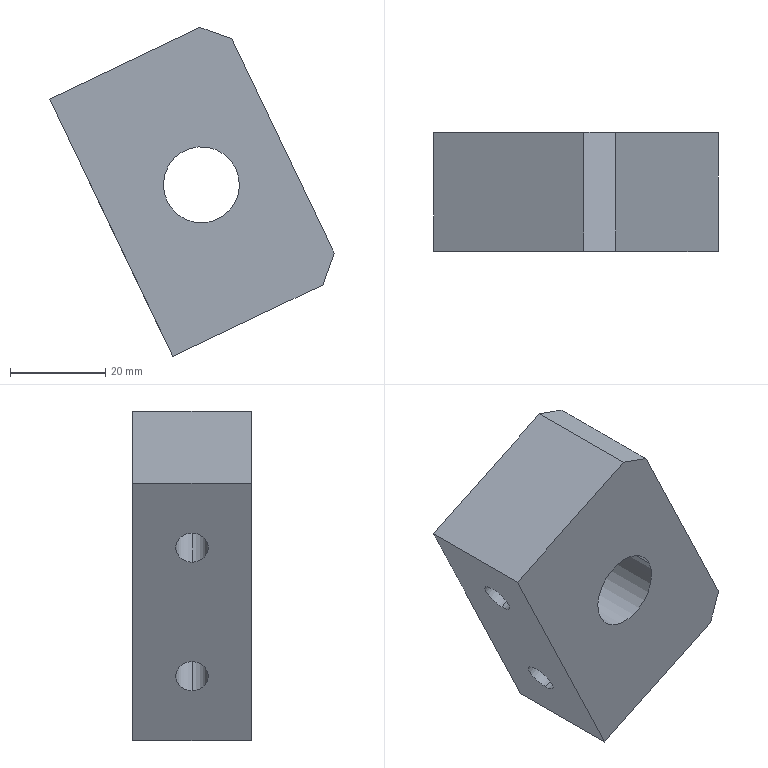Component | SolidWorks | FeedingPressingPlateAdjustmentBlock1-1-1 | 1 solid | 18 faces | box 59.83 x 25 x 69.23 mm | volume 52864 mm3 | plane 8 | cylinder 6 | cone 4 | commonest cylinder face diameters 6.8 x4 16 x2
build123d program:
from build123d import *

# Parameters (mm, degrees)
SKETCH1_W              = 60
SKETCH1_H              = 25
BOSS_EXTRUDE1_DEPTH    = 40
M8_TAPPED_HOLE1_D      = 6.8
M8_TAPPED_HOLE1_DEPTH  = 19.75
M8_TAPPED_HOLE1_TIP    = 2.043
M16_TAPPED_HOLE1_D     = 16
M16_TAPPED_HOLE1_DEPTH = 38
M16_TAPPED_HOLE1_TIP   = 4.807
CHAMFER1_SIZE          = 5


with BuildPart() as part:
    # Sketch1 → Boss-Extrude1 (new body)
    with BuildSketch(Plane.XY):
        with Locations((30, 12.5)):
            Rectangle(SKETCH1_W, SKETCH1_H)
    extrude(amount=BOSS_EXTRUDE1_DEPTH)

    # M8 Tapped Hole1
    with Locations(Plane(origin=(45, 12.5, 0), x_dir=(-1, 0, 0), z_dir=(0, 0, -1))):
        with Locations((0, 0), (30, 0)):
            Hole(M8_TAPPED_HOLE1_D / 2, depth=M8_TAPPED_HOLE1_DEPTH)
            with Locations((0, 0, -(M8_TAPPED_HOLE1_DEPTH + M8_TAPPED_HOLE1_TIP / 2))):  # 118° drill point
                Cone(0, M8_TAPPED_HOLE1_D / 2, M8_TAPPED_HOLE1_TIP, mode=Mode.SUBTRACT)

    # M16 Tapped Hole1
    with Locations(Plane(origin=(30, 25, 21), x_dir=(0, 0, 1), z_dir=(0, 1, 0))):
        with Locations((0, 0)):
            Hole(M16_TAPPED_HOLE1_D / 2, depth=M16_TAPPED_HOLE1_DEPTH)
            with Locations((0, 0, -(M16_TAPPED_HOLE1_DEPTH + M16_TAPPED_HOLE1_TIP / 2))):  # 118° drill point
                Cone(0, M16_TAPPED_HOLE1_D / 2, M16_TAPPED_HOLE1_TIP, mode=Mode.SUBTRACT)

    # Chamfer1
    chamfer1_edges = [part.edges().sort_by_distance(p)[0] for p in [
        (60, 12.5, 40),
        (0, 12.5, 40),
    ]]
    chamfer(chamfer1_edges, length=CHAMFER1_SIZE)


solid = part.part

# Placed as in the assembly
solid = solid.moved(Location((-27.022, 360, 606.201), (0, 64.419, 0)))
STEP:
#1=COLOUR_RGB('',0.7922,0.8196,0.9333);
#2=FILL_AREA_STYLE_COLOUR('',#1);
#3=FILL_AREA_STYLE('',(#2));
#4=SURFACE_STYLE_FILL_AREA(#3);
#5=SURFACE_SIDE_STYLE('',(#4));
#6=SURFACE_STYLE_USAGE(.BOTH.,#5);
#7=PRESENTATION_STYLE_ASSIGNMENT((#6));
#8=CARTESIAN_POINT('',(-0.09223,14.173,23.022));
#9=VERTEX_POINT('',#8);
#10=CARTESIAN_POINT('',(0.4759,14.173,23.294));
#11=VERTEX_POINT('',#10);
#12=CARTESIAN_POINT('',(0.1919,14.173,23.158));
#13=DIRECTION('',(0.,1.,-0.));
#14=DIRECTION('',(0.902,0.,0.4318));
#15=AXIS2_PLACEMENT_3D('',#12,#13,#14);
#16=CIRCLE('',#15,0.315);
#17=EDGE_CURVE('',#9,#11,#16,.T.);
#18=ORIENTED_EDGE('',*,*,#17,.F.);
#19=CARTESIAN_POINT('',(-0.09223,15.157,23.022));
#20=VERTEX_POINT('',#19);
#21=CARTESIAN_POINT('',(-0.09223,15.157,23.022));
#22=DIRECTION('',(0.,1.,-0.));
#23=VECTOR('',#22,39.37);
#24=LINE('',#21,#23);
#25=EDGE_CURVE('',#9,#20,#24,.T.);
#26=ORIENTED_EDGE('',*,*,#25,.T.);
#27=CARTESIAN_POINT('',(0.4759,15.157,23.294));
#28=VERTEX_POINT('',#27);
#29=CARTESIAN_POINT('',(0.1919,15.157,23.158));
#30=DIRECTION('',(0.,1.,-0.));
#31=DIRECTION('',(0.902,0.,0.4318));
#32=AXIS2_PLACEMENT_3D('',#29,#30,#31);
#33=CIRCLE('',#32,0.315);
#34=EDGE_CURVE('',#20,#28,#33,.T.);
#35=ORIENTED_EDGE('',*,*,#34,.T.);
#36=CARTESIAN_POINT('',(0.4759,15.157,23.294));
#37=DIRECTION('',(0.,1.,-0.));
#38=VECTOR('',#37,39.37);
#39=LINE('',#36,#38);
#40=EDGE_CURVE('',#11,#28,#39,.T.);
#41=ORIENTED_EDGE('',*,*,#40,.F.);
#42=EDGE_LOOP('',(#18,#26,#35,#41));
#43=FACE_OUTER_BOUND('',#42,.T.);
#44=CARTESIAN_POINT('',(0.1919,15.157,23.158));
#45=DIRECTION('',(0.,1.,-0.));
#46=DIRECTION('',(0.902,0.,0.4318));
#47=AXIS2_PLACEMENT_3D('',#44,#45,#46);
#48=CYLINDRICAL_SURFACE('',#47,0.315);
#49=ADVANCED_FACE('',(#43),#48,.F.);
#50=CARTESIAN_POINT('',(0.4603,14.665,22.483));
#51=VERTEX_POINT('',#50);
#52=CARTESIAN_POINT('',(0.3447,14.665,22.725));
#53=VERTEX_POINT('',#52);
#54=CARTESIAN_POINT('',(0.4025,14.665,22.604));
#55=DIRECTION('',(-0.902,0.,-0.4318));
#56=DIRECTION('',(-0.4318,0.,0.902));
#57=AXIS2_PLACEMENT_3D('',#54,#55,#56);
#58=CIRCLE('',#57,0.1339);
#59=EDGE_CURVE('',#51,#53,#58,.T.);
#60=ORIENTED_EDGE('',*,*,#59,.F.);
#61=CARTESIAN_POINT('',(-0.2411,14.665,22.147));
#62=VERTEX_POINT('',#61);
#63=CARTESIAN_POINT('',(-0.2411,14.665,22.147));
#64=DIRECTION('',(-0.902,0.,-0.4318));
#65=VECTOR('',#64,39.37);
#66=LINE('',#63,#65);
#67=EDGE_CURVE('',#51,#62,#66,.T.);
#68=ORIENTED_EDGE('',*,*,#67,.T.);
#69=CARTESIAN_POINT('',(-0.3567,14.665,22.389));
#70=VERTEX_POINT('',#69);
#71=CARTESIAN_POINT('',(-0.2989,14.665,22.268));
#72=DIRECTION('',(-0.902,0.,-0.4318));
#73=DIRECTION('',(-0.4318,0.,0.902));
#74=AXIS2_PLACEMENT_3D('',#71,#72,#73);
#75=CIRCLE('',#74,0.1339);
#76=EDGE_CURVE('',#62,#70,#75,.T.);
#77=ORIENTED_EDGE('',*,*,#76,.T.);
#78=CARTESIAN_POINT('',(-0.3567,14.665,22.389));
#79=DIRECTION('',(-0.902,0.,-0.4318));
#80=VECTOR('',#79,39.37);
#81=LINE('',#78,#80);
#82=EDGE_CURVE('',#53,#70,#81,.T.);
#83=ORIENTED_EDGE('',*,*,#82,.F.);
#84=EDGE_LOOP('',(#60,#68,#77,#83));
#85=FACE_OUTER_BOUND('',#84,.T.);
#86=CARTESIAN_POINT('',(-0.2989,14.665,22.268));
#87=DIRECTION('',(-0.902,0.,-0.4318));
#88=DIRECTION('',(-0.4318,0.,0.902));
#89=AXIS2_PLACEMENT_3D('',#86,#87,#88);
#90=CYLINDRICAL_SURFACE('',#89,0.1339);
#91=ADVANCED_FACE('',(#85),#90,.F.);
#92=CARTESIAN_POINT('',(0.475,14.665,22.639));
#93=VERTEX_POINT('',#92);
#94=CARTESIAN_POINT('',(0.3447,14.665,22.725));
#95=DIRECTION('',(-0.8347,0.,0.5508));
#96=VECTOR('',#95,39.37);
#97=LINE('',#94,#96);
#98=EDGE_CURVE('',#93,#53,#97,.T.);
#99=ORIENTED_EDGE('',*,*,#98,.F.);
#100=CARTESIAN_POINT('',(0.4603,14.665,22.483));
#101=DIRECTION('',(-0.09444,-0.,-0.9955));
#102=VECTOR('',#101,39.37);
#103=LINE('',#100,#102);
#104=EDGE_CURVE('',#93,#51,#103,.T.);
#105=ORIENTED_EDGE('',*,*,#104,.T.);
#106=ORIENTED_EDGE('',*,*,#59,.T.);
#107=EDGE_LOOP('',(#99,#105,#106));
#108=FACE_OUTER_BOUND('',#107,.T.);
#109=CARTESIAN_POINT('',(0.4025,14.665,22.604));
#110=DIRECTION('',(-0.902,0.,-0.4318));
#111=DIRECTION('',(-0.4318,0.,0.902));
#112=AXIS2_PLACEMENT_3D('',#109,#110,#111);
#113=CONICAL_SURFACE('',#112,0.1339,1.03);
#114=ADVANCED_FACE('',(#108),#113,.F.);
#115=CARTESIAN_POINT('',(-0.04972,14.665,23.549));
#116=VERTEX_POINT('',#115);
#117=CARTESIAN_POINT('',(-0.1653,14.665,23.79));
#118=VERTEX_POINT('',#117);
#119=CARTESIAN_POINT('',(-0.1075,14.665,23.669));
#120=DIRECTION('',(-0.902,0.,-0.4318));
#121=DIRECTION('',(-0.4318,0.,0.902));
#122=AXIS2_PLACEMENT_3D('',#119,#120,#121);
#123=CIRCLE('',#122,0.1339);
#124=EDGE_CURVE('',#116,#118,#123,.T.);
#125=ORIENTED_EDGE('',*,*,#124,.F.);
#126=CARTESIAN_POINT('',(-0.7511,14.665,23.213));
#127=VERTEX_POINT('',#126);
#128=CARTESIAN_POINT('',(-0.7511,14.665,23.213));
#129=DIRECTION('',(-0.902,0.,-0.4318));
#130=VECTOR('',#129,39.37);
#131=LINE('',#128,#130);
#132=EDGE_CURVE('',#116,#127,#131,.T.);
#133=ORIENTED_EDGE('',*,*,#132,.T.);
#134=CARTESIAN_POINT('',(-0.8667,14.665,23.454));
#135=VERTEX_POINT('',#134);
#136=CARTESIAN_POINT('',(-0.8089,14.665,23.334));
#137=DIRECTION('',(-0.902,0.,-0.4318));
#138=DIRECTION('',(-0.4318,0.,0.902));
#139=AXIS2_PLACEMENT_3D('',#136,#137,#138);
#140=CIRCLE('',#139,0.1339);
#141=EDGE_CURVE('',#127,#135,#140,.T.);
#142=ORIENTED_EDGE('',*,*,#141,.T.);
#143=CARTESIAN_POINT('',(-0.8667,14.665,23.454));
#144=DIRECTION('',(-0.902,0.,-0.4318));
#145=VECTOR('',#144,39.37);
#146=LINE('',#143,#145);
#147=EDGE_CURVE('',#118,#135,#146,.T.);
#148=ORIENTED_EDGE('',*,*,#147,.F.);
#149=EDGE_LOOP('',(#125,#133,#142,#148));
#150=FACE_OUTER_BOUND('',#149,.T.);
#151=CARTESIAN_POINT('',(-0.8089,14.665,23.334));
#152=DIRECTION('',(-0.902,0.,-0.4318));
#153=DIRECTION('',(-0.4318,0.,0.902));
#154=AXIS2_PLACEMENT_3D('',#151,#152,#153);
#155=CYLINDRICAL_SURFACE('',#154,0.1339);
#156=ADVANCED_FACE('',(#150),#155,.F.);
#157=CARTESIAN_POINT('',(-0.03498,14.665,23.704));
#158=VERTEX_POINT('',#157);
#159=CARTESIAN_POINT('',(-0.1653,14.665,23.79));
#160=DIRECTION('',(-0.8347,0.,0.5508));
#161=VECTOR('',#160,39.37);
#162=LINE('',#159,#161);
#163=EDGE_CURVE('',#158,#118,#162,.T.);
#164=ORIENTED_EDGE('',*,*,#163,.F.);
#165=CARTESIAN_POINT('',(-0.04972,14.665,23.549));
#166=DIRECTION('',(-0.09444,-0.,-0.9955));
#167=VECTOR('',#166,39.37);
#168=LINE('',#165,#167);
#169=EDGE_CURVE('',#158,#116,#168,.T.);
#170=ORIENTED_EDGE('',*,*,#169,.T.);
#171=ORIENTED_EDGE('',*,*,#124,.T.);
#172=EDGE_LOOP('',(#164,#170,#171));
#173=FACE_OUTER_BOUND('',#172,.T.);
#174=CARTESIAN_POINT('',(-0.1075,14.665,23.669));
#175=DIRECTION('',(-0.902,0.,-0.4318));
#176=DIRECTION('',(-0.4318,0.,0.902));
#177=AXIS2_PLACEMENT_3D('',#174,#175,#176);
#178=CONICAL_SURFACE('',#177,0.1339,1.03);
#179=ADVANCED_FACE('',(#173),#178,.F.);
#180=CARTESIAN_POINT('',(0.179,14.173,24.461));
#181=VERTEX_POINT('',#180);
#182=CARTESIAN_POINT('',(-1.064,14.173,23.866));
#183=VERTEX_POINT('',#182);
#184=CARTESIAN_POINT('',(0.3566,14.173,24.546));
#185=DIRECTION('',(-0.902,0.,-0.4318));
#186=VECTOR('',#185,39.37);
#187=LINE('',#184,#186);
#188=EDGE_CURVE('',#181,#183,#187,.T.);
#189=ORIENTED_EDGE('',*,*,#188,.F.);
#190=CARTESIAN_POINT('',(0.179,15.157,24.461));
#191=VERTEX_POINT('',#190);
#192=CARTESIAN_POINT('',(0.179,14.173,24.461));
#193=DIRECTION('',(0.,1.,-0.));
#194=VECTOR('',#193,39.37);
#195=LINE('',#192,#194);
#196=EDGE_CURVE('',#181,#191,#195,.T.);
#197=ORIENTED_EDGE('',*,*,#196,.T.);
#198=CARTESIAN_POINT('',(-1.064,15.157,23.866));
#199=VERTEX_POINT('',#198);
#200=CARTESIAN_POINT('',(0.3566,15.157,24.546));
#201=DIRECTION('',(-0.902,0.,-0.4318));
#202=VECTOR('',#201,39.37);
#203=LINE('',#200,#202);
#204=EDGE_CURVE('',#191,#199,#203,.T.);
#205=ORIENTED_EDGE('',*,*,#204,.T.);
#206=CARTESIAN_POINT('',(-1.064,14.173,23.866));
#207=DIRECTION('',(-0.,-1.,0.));
#208=VECTOR('',#207,39.37);
#209=LINE('',#206,#208);
#210=EDGE_CURVE('',#199,#183,#209,.T.);
#211=ORIENTED_EDGE('',*,*,#210,.T.);
#212=EDGE_LOOP('',(#189,#197,#205,#211));
#213=FACE_OUTER_BOUND('',#212,.T.);
#214=CARTESIAN_POINT('',(0.3566,14.173,24.546));
#215=DIRECTION('',(0.4318,-0.,-0.902));
#216=DIRECTION('',(-0.902,0.,-0.4318));
#217=AXIS2_PLACEMENT_3D('',#214,#215,#216);
#218=PLANE('',#217);
#219=ADVANCED_FACE('',(#213),#218,.F.);
#220=CARTESIAN_POINT('',(0.1919,14.173,23.158));
#221=DIRECTION('',(0.,1.,-0.));
#222=DIRECTION('',(0.902,0.,0.4318));
#223=AXIS2_PLACEMENT_3D('',#220,#221,#222);
#224=CIRCLE('',#223,0.315);
#225=EDGE_CURVE('',#11,#9,#224,.T.);
#226=ORIENTED_EDGE('',*,*,#225,.T.);
#227=ORIENTED_EDGE('',*,*,#17,.T.);
#228=EDGE_LOOP('',(#226,#227));
#229=FACE_BOUND('',#228,.T.);
#230=CARTESIAN_POINT('',(1.199,14.173,22.33));
#231=VERTEX_POINT('',#230);
#232=CARTESIAN_POINT('',(-0.04389,14.173,21.736));
#233=VERTEX_POINT('',#232);
#234=CARTESIAN_POINT('',(1.377,14.173,22.415));
#235=DIRECTION('',(-0.902,0.,-0.4318));
#236=VECTOR('',#235,39.37);
#237=LINE('',#234,#236);
#238=EDGE_CURVE('',#231,#233,#237,.T.);
#239=ORIENTED_EDGE('',*,*,#238,.F.);
#240=CARTESIAN_POINT('',(1.292,14.173,22.593));
#241=VERTEX_POINT('',#240);
#242=CARTESIAN_POINT('',(1.292,14.173,22.593));
#243=DIRECTION('',(0.3325,0.,0.9431));
#244=VECTOR('',#243,39.37);
#245=LINE('',#242,#244);
#246=EDGE_CURVE('',#231,#241,#245,.T.);
#247=ORIENTED_EDGE('',*,*,#246,.T.);
#248=CARTESIAN_POINT('',(0.4416,14.173,24.369));
#249=VERTEX_POINT('',#248);
#250=CARTESIAN_POINT('',(0.3566,14.173,24.546));
#251=DIRECTION('',(0.4318,-0.,-0.902));
#252=VECTOR('',#251,39.37);
#253=LINE('',#250,#252);
#254=EDGE_CURVE('',#249,#241,#253,.T.);
#255=ORIENTED_EDGE('',*,*,#254,.F.);
#256=CARTESIAN_POINT('',(0.4416,14.173,24.369));
#257=DIRECTION('',(-0.9431,0.,0.3325));
#258=VECTOR('',#257,39.37);
#259=LINE('',#256,#258);
#260=EDGE_CURVE('',#249,#181,#259,.T.);
#261=ORIENTED_EDGE('',*,*,#260,.T.);
#262=ORIENTED_EDGE('',*,*,#188,.T.);
#263=CARTESIAN_POINT('',(-1.064,14.173,23.866));
#264=DIRECTION('',(0.4318,-0.,-0.902));
#265=VECTOR('',#264,39.37);
#266=LINE('',#263,#265);
#267=EDGE_CURVE('',#183,#233,#266,.T.);
#268=ORIENTED_EDGE('',*,*,#267,.T.);
#269=EDGE_LOOP('',(#239,#247,#255,#261,#262,#268));
#270=FACE_OUTER_BOUND('',#269,.T.);
#271=CARTESIAN_POINT('',(0.3566,14.173,24.546));
#272=DIRECTION('',(0.,1.,-0.));
#273=DIRECTION('',(0.902,-0.,0.4318));
#274=AXIS2_PLACEMENT_3D('',#271,#272,#273);
#275=PLANE('',#274);
#276=ADVANCED_FACE('',(#229,#270),#275,.F.);
#277=CARTESIAN_POINT('',(1.199,15.157,22.33));
#278=VERTEX_POINT('',#277);
#279=CARTESIAN_POINT('',(-0.04389,15.157,21.736));
#280=VERTEX_POINT('',#279);
#281=CARTESIAN_POINT('',(1.377,15.157,22.415));
#282=DIRECTION('',(-0.902,0.,-0.4318));
#283=VECTOR('',#282,39.37);
#284=LINE('',#281,#283);
#285=EDGE_CURVE('',#278,#280,#284,.T.);
#286=ORIENTED_EDGE('',*,*,#285,.F.);
#287=CARTESIAN_POINT('',(1.199,14.173,22.33));
#288=DIRECTION('',(-0.,-1.,0.));
#289=VECTOR('',#288,39.37);
#290=LINE('',#287,#289);
#291=EDGE_CURVE('',#278,#231,#290,.T.);
#292=ORIENTED_EDGE('',*,*,#291,.T.);
#293=ORIENTED_EDGE('',*,*,#238,.T.);
#294=CARTESIAN_POINT('',(-0.04389,14.173,21.736));
#295=DIRECTION('',(0.,1.,-0.));
#296=VECTOR('',#295,39.37);
#297=LINE('',#294,#296);
#298=EDGE_CURVE('',#233,#280,#297,.T.);
#299=ORIENTED_EDGE('',*,*,#298,.T.);
#300=EDGE_LOOP('',(#286,#292,#293,#299));
#301=FACE_OUTER_BOUND('',#300,.T.);
#302=CARTESIAN_POINT('',(1.377,14.173,22.415));
#303=DIRECTION('',(-0.4318,0.,0.902));
#304=DIRECTION('',(0.902,-0.,0.4318));
#305=AXIS2_PLACEMENT_3D('',#302,#303,#304);
#306=PLANE('',#305);
#307=ADVANCED_FACE('',(#301),#306,.F.);
#308=CARTESIAN_POINT('',(0.1919,15.157,23.158));
#309=DIRECTION('',(0.,1.,-0.));
#310=DIRECTION('',(0.902,0.,0.4318));
#311=AXIS2_PLACEMENT_3D('',#308,#309,#310);
#312=CIRCLE('',#311,0.315);
#313=EDGE_CURVE('',#28,#20,#312,.T.);
#314=ORIENTED_EDGE('',*,*,#313,.F.);
#315=ORIENTED_EDGE('',*,*,#34,.F.);
#316=EDGE_LOOP('',(#314,#315));
#317=FACE_BOUND('',#316,.T.);
#318=CARTESIAN_POINT('',(1.292,15.157,22.593));
#319=VERTEX_POINT('',#318);
#320=CARTESIAN_POINT('',(0.4416,15.157,24.369));
#321=VERTEX_POINT('',#320);
#322=CARTESIAN_POINT('',(0.3566,15.157,24.546));
#323=DIRECTION('',(-0.4318,0.,0.902));
#324=VECTOR('',#323,39.37);
#325=LINE('',#322,#324);
#326=EDGE_CURVE('',#319,#321,#325,.T.);
#327=ORIENTED_EDGE('',*,*,#326,.F.);
#328=CARTESIAN_POINT('',(1.292,15.157,22.593));
#329=DIRECTION('',(-0.3325,-0.,-0.9431));
#330=VECTOR('',#329,39.37);
#331=LINE('',#328,#330);
#332=EDGE_CURVE('',#319,#278,#331,.T.);
#333=ORIENTED_EDGE('',*,*,#332,.T.);
#334=ORIENTED_EDGE('',*,*,#285,.T.);
#335=CARTESIAN_POINT('',(-1.064,15.157,23.866));
#336=DIRECTION('',(-0.4318,0.,0.902));
#337=VECTOR('',#336,39.37);
#338=LINE('',#335,#337);
#339=EDGE_CURVE('',#280,#199,#338,.T.);
#340=ORIENTED_EDGE('',*,*,#339,.T.);
#341=ORIENTED_EDGE('',*,*,#204,.F.);
#342=CARTESIAN_POINT('',(0.4416,15.157,24.369));
#343=DIRECTION('',(0.9431,-0.,-0.3325));
#344=VECTOR('',#343,39.37);
#345=LINE('',#342,#344);
#346=EDGE_CURVE('',#191,#321,#345,.T.);
#347=ORIENTED_EDGE('',*,*,#346,.T.);
#348=EDGE_LOOP('',(#327,#333,#334,#340,#341,#347));
#349=FACE_OUTER_BOUND('',#348,.T.);
#350=CARTESIAN_POINT('',(0.3566,15.157,24.546));
#351=DIRECTION('',(-0.,-1.,0.));
#352=DIRECTION('',(-0.902,0.,-0.4318));
#353=AXIS2_PLACEMENT_3D('',#350,#351,#352);
#354=PLANE('',#353);
#355=ADVANCED_FACE('',(#317,#349),#354,.F.);
#356=ORIENTED_EDGE('',*,*,#254,.T.);
#357=CARTESIAN_POINT('',(1.292,14.173,22.593));
#358=DIRECTION('',(0.,1.,-0.));
#359=VECTOR('',#358,39.37);
#360=LINE('',#357,#359);
#361=EDGE_CURVE('',#241,#319,#360,.T.);
#362=ORIENTED_EDGE('',*,*,#361,.T.);
#363=ORIENTED_EDGE('',*,*,#326,.T.);
#364=CARTESIAN_POINT('',(0.4416,14.173,24.369));
#365=DIRECTION('',(-0.,-1.,0.));
#366=VECTOR('',#365,39.37);
#367=LINE('',#364,#366);
#368=EDGE_CURVE('',#321,#249,#367,.T.);
#369=ORIENTED_EDGE('',*,*,#368,.T.);
#370=EDGE_LOOP('',(#356,#362,#363,#369));
#371=FACE_OUTER_BOUND('',#370,.T.);
#372=CARTESIAN_POINT('',(0.3566,14.173,24.546));
#373=DIRECTION('',(-0.902,0.,-0.4318));
#374=DIRECTION('',(-0.4318,0.,0.902));
#375=AXIS2_PLACEMENT_3D('',#372,#373,#374);
#376=PLANE('',#375);
#377=ADVANCED_FACE('',(#371),#376,.F.);
#378=CARTESIAN_POINT('',(-0.2989,14.665,22.268));
#379=DIRECTION('',(-0.902,0.,-0.4318));
#380=DIRECTION('',(-0.4318,0.,0.902));
#381=AXIS2_PLACEMENT_3D('',#378,#379,#380);
#382=CIRCLE('',#381,0.1339);
#383=EDGE_CURVE('',#70,#62,#382,.T.);
#384=ORIENTED_EDGE('',*,*,#383,.F.);
#385=ORIENTED_EDGE('',*,*,#76,.F.);
#386=EDGE_LOOP('',(#384,#385));
#387=FACE_BOUND('',#386,.T.);
#388=CARTESIAN_POINT('',(-0.8089,14.665,23.334));
#389=DIRECTION('',(-0.902,0.,-0.4318));
#390=DIRECTION('',(-0.4318,0.,0.902));
#391=AXIS2_PLACEMENT_3D('',#388,#389,#390);
#392=CIRCLE('',#391,0.1339);
#393=EDGE_CURVE('',#135,#127,#392,.T.);
#394=ORIENTED_EDGE('',*,*,#393,.F.);
#395=ORIENTED_EDGE('',*,*,#141,.F.);
#396=EDGE_LOOP('',(#394,#395));
#397=FACE_BOUND('',#396,.T.);
#398=ORIENTED_EDGE('',*,*,#210,.F.);
#399=ORIENTED_EDGE('',*,*,#339,.F.);
#400=ORIENTED_EDGE('',*,*,#298,.F.);
#401=ORIENTED_EDGE('',*,*,#267,.F.);
#402=EDGE_LOOP('',(#398,#399,#400,#401));
#403=FACE_OUTER_BOUND('',#402,.T.);
#404=CARTESIAN_POINT('',(-1.064,14.173,23.866));
#405=DIRECTION('',(-0.902,0.,-0.4318));
#406=DIRECTION('',(-0.4318,0.,0.902));
#407=AXIS2_PLACEMENT_3D('',#404,#405,#406);
#408=PLANE('',#407);
#409=ADVANCED_FACE('',(#387,#397,#403),#408,.T.);
#410=ORIENTED_EDGE('',*,*,#169,.F.);
#411=ORIENTED_EDGE('',*,*,#163,.T.);
#412=CARTESIAN_POINT('',(-0.1075,14.665,23.669));
#413=DIRECTION('',(-0.902,0.,-0.4318));
#414=DIRECTION('',(-0.4318,0.,0.902));
#415=AXIS2_PLACEMENT_3D('',#412,#413,#414);
#416=CIRCLE('',#415,0.1339);
#417=EDGE_CURVE('',#118,#116,#416,.T.);
#418=ORIENTED_EDGE('',*,*,#417,.T.);
#419=EDGE_LOOP('',(#410,#411,#418));
#420=FACE_OUTER_BOUND('',#419,.T.);
#421=CARTESIAN_POINT('',(-0.1075,14.665,23.669));
#422=DIRECTION('',(-0.902,0.,-0.4318));
#423=DIRECTION('',(-0.4318,0.,0.902));
#424=AXIS2_PLACEMENT_3D('',#421,#422,#423);
#425=CONICAL_SURFACE('',#424,0.1339,1.03);
#426=ADVANCED_FACE('',(#420),#425,.F.);
#427=ORIENTED_EDGE('',*,*,#132,.F.);
#428=ORIENTED_EDGE('',*,*,#417,.F.);
#429=ORIENTED_EDGE('',*,*,#147,.T.);
#430=ORIENTED_EDGE('',*,*,#393,.T.);
#431=EDGE_LOOP('',(#427,#428,#429,#430));
#432=FACE_OUTER_BOUND('',#431,.T.);
#433=CARTESIAN_POINT('',(-0.8089,14.665,23.334));
#434=DIRECTION('',(-0.902,0.,-0.4318));
#435=DIRECTION('',(-0.4318,0.,0.902));
#436=AXIS2_PLACEMENT_3D('',#433,#434,#435);
#437=CYLINDRICAL_SURFACE('',#436,0.1339);
#438=ADVANCED_FACE('',(#432),#437,.F.);
#439=ORIENTED_EDGE('',*,*,#104,.F.);
#440=ORIENTED_EDGE('',*,*,#98,.T.);
#441=CARTESIAN_POINT('',(0.4025,14.665,22.604));
#442=DIRECTION('',(-0.902,0.,-0.4318));
#443=DIRECTION('',(-0.4318,0.,0.902));
#444=AXIS2_PLACEMENT_3D('',#441,#442,#443);
#445=CIRCLE('',#444,0.1339);
#446=EDGE_CURVE('',#53,#51,#445,.T.);
#447=ORIENTED_EDGE('',*,*,#446,.T.);
#448=EDGE_LOOP('',(#439,#440,#447));
#449=FACE_OUTER_BOUND('',#448,.T.);
#450=CARTESIAN_POINT('',(0.4025,14.665,22.604));
#451=DIRECTION('',(-0.902,0.,-0.4318));
#452=DIRECTION('',(-0.4318,0.,0.902));
#453=AXIS2_PLACEMENT_3D('',#450,#451,#452);
#454=CONICAL_SURFACE('',#453,0.1339,1.03);
#455=ADVANCED_FACE('',(#449),#454,.F.);
#456=ORIENTED_EDGE('',*,*,#67,.F.);
#457=ORIENTED_EDGE('',*,*,#446,.F.);
#458=ORIENTED_EDGE('',*,*,#82,.T.);
#459=ORIENTED_EDGE('',*,*,#383,.T.);
#460=EDGE_LOOP('',(#456,#457,#458,#459));
#461=FACE_OUTER_BOUND('',#460,.T.);
#462=CARTESIAN_POINT('',(-0.2989,14.665,22.268));
#463=DIRECTION('',(-0.902,0.,-0.4318));
#464=DIRECTION('',(-0.4318,0.,0.902));
#465=AXIS2_PLACEMENT_3D('',#462,#463,#464);
#466=CYLINDRICAL_SURFACE('',#465,0.1339);
#467=ADVANCED_FACE('',(#461),#466,.F.);
#468=ORIENTED_EDGE('',*,*,#25,.F.);
#469=ORIENTED_EDGE('',*,*,#225,.F.);
#470=ORIENTED_EDGE('',*,*,#40,.T.);
#471=ORIENTED_EDGE('',*,*,#313,.T.);
#472=EDGE_LOOP('',(#468,#469,#470,#471));
#473=FACE_OUTER_BOUND('',#472,.T.);
#474=CARTESIAN_POINT('',(0.1919,15.157,23.158));
#475=DIRECTION('',(0.,1.,-0.));
#476=DIRECTION('',(0.902,0.,0.4318));
#477=AXIS2_PLACEMENT_3D('',#474,#475,#476);
#478=CYLINDRICAL_SURFACE('',#477,0.315);
#479=ADVANCED_FACE('',(#473),#478,.F.);
#480=ORIENTED_EDGE('',*,*,#246,.F.);
#481=ORIENTED_EDGE('',*,*,#291,.F.);
#482=ORIENTED_EDGE('',*,*,#332,.F.);
#483=ORIENTED_EDGE('',*,*,#361,.F.);
#484=EDGE_LOOP('',(#480,#481,#482,#483));
#485=FACE_OUTER_BOUND('',#484,.T.);
#486=CARTESIAN_POINT('',(1.292,14.173,22.593));
#487=DIRECTION('',(-0.9431,0.,0.3325));
#488=DIRECTION('',(0.,1.,-0.));
#489=AXIS2_PLACEMENT_3D('',#486,#487,#488);
#490=PLANE('',#489);
#491=ADVANCED_FACE('',(#485),#490,.F.);
#492=ORIENTED_EDGE('',*,*,#346,.F.);
#493=ORIENTED_EDGE('',*,*,#196,.F.);
#494=ORIENTED_EDGE('',*,*,#260,.F.);
#495=ORIENTED_EDGE('',*,*,#368,.F.);
#496=EDGE_LOOP('',(#492,#493,#494,#495));
#497=FACE_OUTER_BOUND('',#496,.T.);
#498=CARTESIAN_POINT('',(0.4416,14.173,24.369));
#499=DIRECTION('',(-0.3325,-0.,-0.9431));
#500=DIRECTION('',(-0.,-1.,0.));
#501=AXIS2_PLACEMENT_3D('',#498,#499,#500);
#502=PLANE('',#501);
#503=ADVANCED_FACE('',(#497),#502,.F.);
#504=CLOSED_SHELL('',(#49,#91,#114,#156,#179,#219,#276,#307,#355,#377,#409,#426,#438,#455,#467,#479,#491,#503));
#505=MANIFOLD_SOLID_BREP('',#504);
#506=STYLED_ITEM('',(#7),#505);
#507=(LENGTH_UNIT()NAMED_UNIT(*)SI_UNIT($,.METRE.));
#508=LENGTH_MEASURE_WITH_UNIT(LENGTH_MEASURE(0.0254),#507);
#509=DIMENSIONAL_EXPONENTS(1.,0.,0.,0.,0.,0.,0.);
#510=(CONVERSION_BASED_UNIT('',#508)LENGTH_UNIT()NAMED_UNIT(#509));
#511=UNCERTAINTY_MEASURE_WITH_UNIT(LENGTH_MEASURE(0.00001),#510,'','');
#512=(NAMED_UNIT(*)PLANE_ANGLE_UNIT()SI_UNIT($,.RADIAN.));
#513=(NAMED_UNIT(*)SI_UNIT($,.STERADIAN.)SOLID_ANGLE_UNIT());
#514=(GEOMETRIC_REPRESENTATION_CONTEXT(3)GLOBAL_UNCERTAINTY_ASSIGNED_CONTEXT((#511))GLOBAL_UNIT_ASSIGNED_CONTEXT((#510,#512,#513))REPRESENTATION_CONTEXT('',''));
#515=MECHANICAL_DESIGN_GEOMETRIC_PRESENTATION_REPRESENTATION('',(#506),#514);
#516=CARTESIAN_POINT('',(0.,0.,0.));
#517=DIRECTION('',(0.,0.,1.));
#518=DIRECTION('',(1.,0.,0.));
#519=AXIS2_PLACEMENT_3D('',#516,#517,#518);
#520=(LENGTH_UNIT()NAMED_UNIT(*)SI_UNIT($,.METRE.));
#521=LENGTH_MEASURE_WITH_UNIT(LENGTH_MEASURE(0.0254),#520);
#522=DIMENSIONAL_EXPONENTS(1.,0.,0.,0.,0.,0.,0.);
#523=(CONVERSION_BASED_UNIT('',#521)LENGTH_UNIT()NAMED_UNIT(#522));
#524=UNCERTAINTY_MEASURE_WITH_UNIT(LENGTH_MEASURE(0.00001),#523,'','');
#525=(NAMED_UNIT(*)PLANE_ANGLE_UNIT()SI_UNIT($,.RADIAN.));
#526=(NAMED_UNIT(*)SI_UNIT($,.STERADIAN.)SOLID_ANGLE_UNIT());
#527=(GEOMETRIC_REPRESENTATION_CONTEXT(3)GLOBAL_UNCERTAINTY_ASSIGNED_CONTEXT((#524))GLOBAL_UNIT_ASSIGNED_CONTEXT((#523,#525,#526))REPRESENTATION_CONTEXT('',''));
#528=ADVANCED_BREP_SHAPE_REPRESENTATION('',(#505,#519),#527);
#529=PRESENTATION_LAYER_ASSIGNMENT('','',(#506));